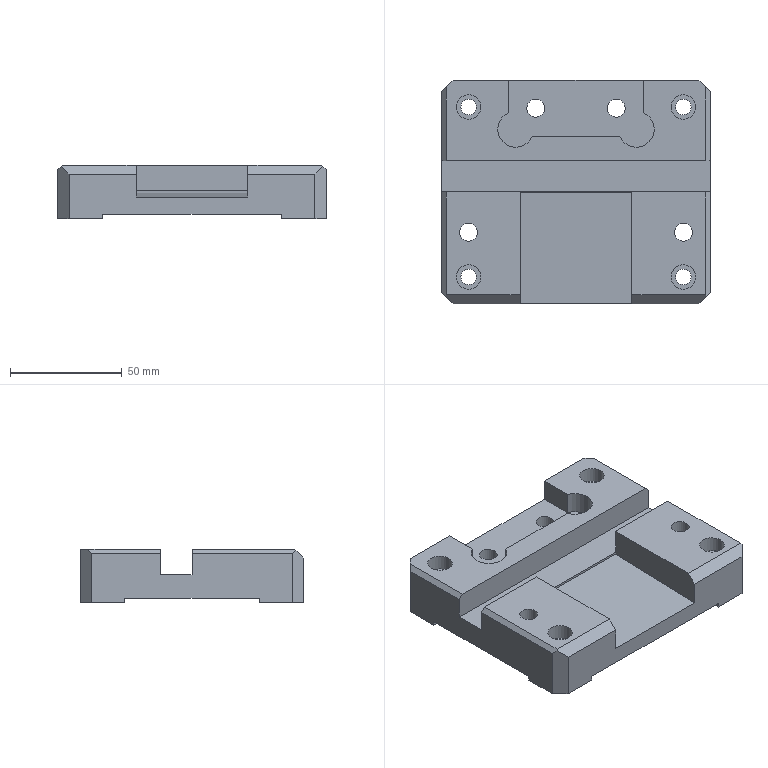Component | NX | 1_BASE_PLATE | 1 solid | 68 faces | volume 186195 mm3 | plane 48 | cylinder 20 | commonest cylinder face diameters 16 x6 11 x6 7 x4 8 x4